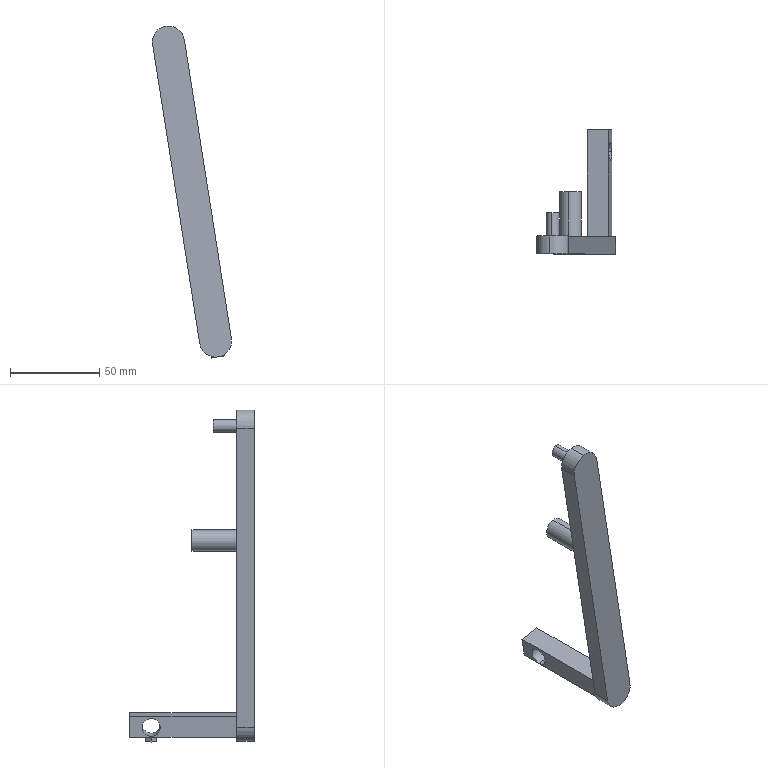Component | SolidWorks | Part2-1 | 1 solid | 27 faces | box 44.44 x 70 x 186.41 mm | volume 44277 mm3 | plane 18 | cylinder 9 | commonest cylinder face diameters 18 x3 10.1 x2 12 x2 7.1 x2
build123d program:
from build123d import *

# Parameters (mm, degrees)
SKETCH1_2_R         = 6
BOSS_EXTRUDE1_DEPTH = 10
SKETCH2_R           = 3.55
BOSS_EXTRUDE2_DEPTH = 13
SKETCH3_R           = 6
BOSS_EXTRUDE3_DEPTH = 25
SKETCH5_R           = 6
BOSS_EXTRUDE5_DEPTH = 20
SKETCH6_W           = 12
SKETCH6_H           = 12
BOSS_EXTRUDE6_DEPTH = 60
BOSS_EXTRUDE7_DEPTH = 3
SKETCH1_R           = 5.05
CUT_EXTRUDE1_DEPTH  = 193.785


with BuildPart() as part:
    # Sketch1_2 → Boss-Extrude1 (new body)
    with BuildSketch(Plane(origin=(0, 0, 0), x_dir=(0, 0, -1), z_dir=(1, 0, 0))):
        with BuildLine():
            Line((0, 9), (170, 9))
            ThreePointArc((170, 9), (179, 0), (170, -9))
            Line((170, -9), (0, -9))
            ThreePointArc((0, -9), (-9, 0), (0, 9))
        make_face()
        with Locations((65, 0)):
            Circle(SKETCH1_2_R, mode=Mode.SUBTRACT)
    extrude(amount=BOSS_EXTRUDE1_DEPTH)

    # Sketch2 → Boss-Extrude2 (add)
    with BuildSketch(Plane(origin=(10, 0, 0), x_dir=(0, 0, -1), z_dir=(1, 0, 0))):
        with Locations(Location((0, 0, 0), (0, 0, 180))):
            Circle(SKETCH2_R)
    extrude(amount=BOSS_EXTRUDE2_DEPTH)



with BuildPart() as body_2:
    # Sketch3 → Boss-Extrude3 (new body)
    with BuildSketch(Plane(origin=(10, 0, 0), x_dir=(0, 0, -1), z_dir=(1, 0, 0))):
        with Locations((65, 0)):
            Circle(SKETCH3_R)
    extrude(amount=BOSS_EXTRUDE3_DEPTH)


with BuildPart() as part_1:
    add(part.part)

    add(body_2.part)  # Boss-Extrude5 merges body 2
    # Sketch5 → Boss-Extrude5 (add)
    with BuildSketch(Plane.ZY):
        with Locations(Location((-65, 0, 0), (0, 0, 180))):
            Circle(SKETCH5_R)
    extrude(amount=-BOSS_EXTRUDE5_DEPTH)

    # Sketch6 → Boss-Extrude6 (add)
    with BuildSketch(Plane(origin=(10, 0, 0), x_dir=(0, 0, -1), z_dir=(1, 0, 0))):
        with Locations((170, 0)):
            Rectangle(SKETCH6_W, SKETCH6_H)
    extrude(amount=BOSS_EXTRUDE6_DEPTH)

    # Sketch7 → Boss-Extrude7 (add)
    with BuildSketch(Plane(origin=(0, 0, -176), x_dir=(-1, 0, 0), z_dir=(0, 0, -1))):
        Polygon((-58, -3.779), (-54.728, -1.889), (-54.728, 1.889), (-58, 3.779), (-61.272, 1.889), (-61.272, -1.889), align=None)
    extrude(amount=BOSS_EXTRUDE7_DEPTH)

    # Sketch1 → Cut-Extrude1 (cut, through all)
    with BuildSketch(Plane.XZ.offset(6)):
        with Locations(Location((57.862, -170.453, 0), (0, 0, 270))):
            Circle(SKETCH1_R)
    extrude(amount=-CUT_EXTRUDE1_DEPTH, mode=Mode.SUBTRACT)


solid = part_1.part

# Placed as in the assembly
solid = solid.moved(Location((679.123, -42.052, -108.622), (0, -8.948, 90)))
STEP:
#1=COLOUR_RGB('',0.7922,0.8196,0.9333);
#2=FILL_AREA_STYLE_COLOUR('',#1);
#3=FILL_AREA_STYLE('',(#2));
#4=SURFACE_STYLE_FILL_AREA(#3);
#5=SURFACE_SIDE_STYLE('',(#4));
#6=SURFACE_STYLE_USAGE(.BOTH.,#5);
#7=PRESENTATION_STYLE_ASSIGNMENT((#6));
#8=CARTESIAN_POINT('',(27.517,0.6224,-10.746));
#9=VERTEX_POINT('',#8);
#10=CARTESIAN_POINT('',(27.578,0.6224,-11.139));
#11=VERTEX_POINT('',#10);
#12=CARTESIAN_POINT('',(27.548,0.6224,-10.942));
#13=DIRECTION('',(0.9878,-0.,0.1555));
#14=DIRECTION('',(0.1555,0.,-0.9878));
#15=AXIS2_PLACEMENT_3D('',#12,#13,#14);
#16=CIRCLE('',#15,0.1988);
#17=EDGE_CURVE('',#9,#11,#16,.T.);
#18=ORIENTED_EDGE('',*,*,#17,.F.);
#19=CARTESIAN_POINT('',(27.983,0.6224,-10.672));
#20=VERTEX_POINT('',#19);
#21=CARTESIAN_POINT('',(27.4,0.6224,-10.764));
#22=DIRECTION('',(0.9878,-0.,0.1555));
#23=VECTOR('',#22,39.37);
#24=LINE('',#21,#23);
#25=EDGE_CURVE('',#9,#20,#24,.T.);
#26=ORIENTED_EDGE('',*,*,#25,.T.);
#27=CARTESIAN_POINT('',(28.045,0.6224,-11.065));
#28=VERTEX_POINT('',#27);
#29=CARTESIAN_POINT('',(28.014,0.6224,-10.869));
#30=DIRECTION('',(0.9878,-0.,0.1555));
#31=DIRECTION('',(0.1555,0.,-0.9878));
#32=AXIS2_PLACEMENT_3D('',#29,#30,#31);
#33=CIRCLE('',#32,0.1988);
#34=EDGE_CURVE('',#20,#28,#33,.T.);
#35=ORIENTED_EDGE('',*,*,#34,.T.);
#36=CARTESIAN_POINT('',(27.462,0.6224,-11.157));
#37=DIRECTION('',(0.9878,-0.,0.1555));
#38=VECTOR('',#37,39.37);
#39=LINE('',#36,#38);
#40=EDGE_CURVE('',#11,#28,#39,.T.);
#41=ORIENTED_EDGE('',*,*,#40,.F.);
#42=EDGE_LOOP('',(#18,#26,#35,#41));
#43=FACE_OUTER_BOUND('',#42,.T.);
#44=CARTESIAN_POINT('',(27.431,0.6224,-10.961));
#45=DIRECTION('',(0.9878,-0.,0.1555));
#46=DIRECTION('',(0.1555,0.,-0.9878));
#47=AXIS2_PLACEMENT_3D('',#44,#45,#46);
#48=CYLINDRICAL_SURFACE('',#47,0.1988);
#49=ADVANCED_FACE('',(#43),#48,.F.);
#50=CARTESIAN_POINT('',(27.172,-0.2776,-7.038));
#51=VERTEX_POINT('',#50);
#52=CARTESIAN_POINT('',(27.098,-0.2776,-6.571));
#53=VERTEX_POINT('',#52);
#54=CARTESIAN_POINT('',(27.135,-0.2776,-6.804));
#55=DIRECTION('',(0.,1.,0.));
#56=DIRECTION('',(0.1555,0.,-0.9878));
#57=AXIS2_PLACEMENT_3D('',#54,#55,#56);
#58=CIRCLE('',#57,0.2362);
#59=EDGE_CURVE('',#51,#53,#58,.T.);
#60=ORIENTED_EDGE('',*,*,#59,.F.);
#61=CARTESIAN_POINT('',(27.172,-1.262,-7.038));
#62=VERTEX_POINT('',#61);
#63=CARTESIAN_POINT('',(27.172,-0.8682,-7.038));
#64=DIRECTION('',(-0.,-1.,-0.));
#65=VECTOR('',#64,39.37);
#66=LINE('',#63,#65);
#67=EDGE_CURVE('',#51,#62,#66,.T.);
#68=ORIENTED_EDGE('',*,*,#67,.T.);
#69=CARTESIAN_POINT('',(27.098,-1.262,-6.571));
#70=VERTEX_POINT('',#69);
#71=CARTESIAN_POINT('',(27.135,-1.262,-6.804));
#72=DIRECTION('',(0.,1.,0.));
#73=DIRECTION('',(0.1555,0.,-0.9878));
#74=AXIS2_PLACEMENT_3D('',#71,#72,#73);
#75=CIRCLE('',#74,0.2362);
#76=EDGE_CURVE('',#62,#70,#75,.T.);
#77=ORIENTED_EDGE('',*,*,#76,.T.);
#78=CARTESIAN_POINT('',(27.098,-0.8682,-6.571));
#79=DIRECTION('',(-0.,-1.,-0.));
#80=VECTOR('',#79,39.37);
#81=LINE('',#78,#80);
#82=EDGE_CURVE('',#53,#70,#81,.T.);
#83=ORIENTED_EDGE('',*,*,#82,.F.);
#84=EDGE_LOOP('',(#60,#68,#77,#83));
#85=FACE_OUTER_BOUND('',#84,.T.);
#86=CARTESIAN_POINT('',(27.135,-0.8682,-6.804));
#87=DIRECTION('',(-0.,-1.,-0.));
#88=DIRECTION('',(-0.1555,0.,0.9878));
#89=AXIS2_PLACEMENT_3D('',#86,#87,#88);
#90=CYLINDRICAL_SURFACE('',#89,0.2362);
#91=ADVANCED_FACE('',(#85),#90,.T.);
#92=CARTESIAN_POINT('',(26.759,-0.7501,-4.415));
#93=VERTEX_POINT('',#92);
#94=CARTESIAN_POINT('',(26.715,-0.7501,-4.138));
#95=VERTEX_POINT('',#94);
#96=CARTESIAN_POINT('',(26.737,-0.7501,-4.276));
#97=DIRECTION('',(0.,1.,0.));
#98=DIRECTION('',(0.1555,0.,-0.9878));
#99=AXIS2_PLACEMENT_3D('',#96,#97,#98);
#100=CIRCLE('',#99,0.1398);
#101=EDGE_CURVE('',#93,#95,#100,.T.);
#102=ORIENTED_EDGE('',*,*,#101,.F.);
#103=CARTESIAN_POINT('',(26.759,-1.262,-4.415));
#104=VERTEX_POINT('',#103);
#105=CARTESIAN_POINT('',(26.759,-0.7501,-4.415));
#106=DIRECTION('',(-0.,-1.,-0.));
#107=VECTOR('',#106,39.37);
#108=LINE('',#105,#107);
#109=EDGE_CURVE('',#93,#104,#108,.T.);
#110=ORIENTED_EDGE('',*,*,#109,.T.);
#111=CARTESIAN_POINT('',(26.715,-1.262,-4.138));
#112=VERTEX_POINT('',#111);
#113=CARTESIAN_POINT('',(26.737,-1.262,-4.276));
#114=DIRECTION('',(0.,1.,0.));
#115=DIRECTION('',(0.1555,0.,-0.9878));
#116=AXIS2_PLACEMENT_3D('',#113,#114,#115);
#117=CIRCLE('',#116,0.1398);
#118=EDGE_CURVE('',#104,#112,#117,.T.);
#119=ORIENTED_EDGE('',*,*,#118,.T.);
#120=CARTESIAN_POINT('',(26.715,-0.7501,-4.138));
#121=DIRECTION('',(-0.,-1.,-0.));
#122=VECTOR('',#121,39.37);
#123=LINE('',#120,#122);
#124=EDGE_CURVE('',#95,#112,#123,.T.);
#125=ORIENTED_EDGE('',*,*,#124,.F.);
#126=EDGE_LOOP('',(#102,#110,#119,#125));
#127=FACE_OUTER_BOUND('',#126,.T.);
#128=CARTESIAN_POINT('',(26.737,-0.7501,-4.276));
#129=DIRECTION('',(-0.,-1.,-0.));
#130=DIRECTION('',(-0.1555,0.,0.9878));
#131=AXIS2_PLACEMENT_3D('',#128,#129,#130);
#132=CYLINDRICAL_SURFACE('',#131,0.1398);
#133=ADVANCED_FACE('',(#127),#132,.T.);
#134=CARTESIAN_POINT('',(26.682,-1.262,-3.926));
#135=VERTEX_POINT('',#134);
#136=CARTESIAN_POINT('',(27.087,-1.262,-4.221));
#137=VERTEX_POINT('',#136);
#138=CARTESIAN_POINT('',(26.737,-1.262,-4.276));
#139=DIRECTION('',(0.,1.,0.));
#140=DIRECTION('',(0.1555,0.,-0.9878));
#141=AXIS2_PLACEMENT_3D('',#138,#139,#140);
#142=CIRCLE('',#141,0.3543);
#143=EDGE_CURVE('',#135,#137,#142,.T.);
#144=ORIENTED_EDGE('',*,*,#143,.F.);
#145=CARTESIAN_POINT('',(26.682,-1.656,-3.926));
#146=VERTEX_POINT('',#145);
#147=CARTESIAN_POINT('',(26.682,-1.262,-3.926));
#148=DIRECTION('',(-0.,-1.,-0.));
#149=VECTOR('',#148,39.37);
#150=LINE('',#147,#149);
#151=EDGE_CURVE('',#135,#146,#150,.T.);
#152=ORIENTED_EDGE('',*,*,#151,.T.);
#153=CARTESIAN_POINT('',(27.087,-1.656,-4.221));
#154=VERTEX_POINT('',#153);
#155=CARTESIAN_POINT('',(26.737,-1.656,-4.276));
#156=DIRECTION('',(0.,1.,0.));
#157=DIRECTION('',(0.1555,0.,-0.9878));
#158=AXIS2_PLACEMENT_3D('',#155,#156,#157);
#159=CIRCLE('',#158,0.3543);
#160=EDGE_CURVE('',#146,#154,#159,.T.);
#161=ORIENTED_EDGE('',*,*,#160,.T.);
#162=CARTESIAN_POINT('',(27.087,-1.262,-4.221));
#163=DIRECTION('',(-0.,-1.,-0.));
#164=VECTOR('',#163,39.37);
#165=LINE('',#162,#164);
#166=EDGE_CURVE('',#137,#154,#165,.T.);
#167=ORIENTED_EDGE('',*,*,#166,.F.);
#168=EDGE_LOOP('',(#144,#152,#161,#167));
#169=FACE_OUTER_BOUND('',#168,.T.);
#170=CARTESIAN_POINT('',(26.737,-1.262,-4.276));
#171=DIRECTION('',(-0.,-1.,-0.));
#172=DIRECTION('',(-0.1555,0.,0.9878));
#173=AXIS2_PLACEMENT_3D('',#170,#171,#172);
#174=CYLINDRICAL_SURFACE('',#173,0.3543);
#175=ADVANCED_FACE('',(#169),#174,.T.);
#176=CARTESIAN_POINT('',(28.048,-1.262,-11.085));
#177=VERTEX_POINT('',#176);
#178=CARTESIAN_POINT('',(27.581,-1.262,-11.158));
#179=VERTEX_POINT('',#178);
#180=CARTESIAN_POINT('',(27.581,-1.262,-11.158));
#181=DIRECTION('',(-0.9878,0.,-0.1555));
#182=VECTOR('',#181,39.37);
#183=LINE('',#180,#182);
#184=EDGE_CURVE('',#177,#179,#183,.T.);
#185=ORIENTED_EDGE('',*,*,#184,.T.);
#186=CARTESIAN_POINT('',(27.581,1.1,-11.158));
#187=VERTEX_POINT('',#186);
#188=CARTESIAN_POINT('',(27.581,1.1,-11.158));
#189=DIRECTION('',(-0.,-1.,-0.));
#190=VECTOR('',#189,39.37);
#191=LINE('',#188,#190);
#192=EDGE_CURVE('',#187,#179,#191,.T.);
#193=ORIENTED_EDGE('',*,*,#192,.F.);
#194=CARTESIAN_POINT('',(28.048,1.1,-11.085));
#195=VERTEX_POINT('',#194);
#196=CARTESIAN_POINT('',(27.581,1.1,-11.158));
#197=DIRECTION('',(-0.9878,0.,-0.1555));
#198=VECTOR('',#197,39.37);
#199=LINE('',#196,#198);
#200=EDGE_CURVE('',#195,#187,#199,.T.);
#201=ORIENTED_EDGE('',*,*,#200,.F.);
#202=CARTESIAN_POINT('',(28.048,1.1,-11.085));
#203=DIRECTION('',(-0.,-1.,-0.));
#204=VECTOR('',#203,39.37);
#205=LINE('',#202,#204);
#206=EDGE_CURVE('',#195,#177,#205,.T.);
#207=ORIENTED_EDGE('',*,*,#206,.T.);
#208=EDGE_LOOP('',(#185,#193,#201,#207));
#209=FACE_OUTER_BOUND('',#208,.T.);
#210=CARTESIAN_POINT('',(27.888,0.7567,-11.11));
#211=VERTEX_POINT('',#210);
#212=CARTESIAN_POINT('',(27.962,0.6279,-11.098));
#213=VERTEX_POINT('',#212);
#214=CARTESIAN_POINT('',(27.888,0.7567,-11.11));
#215=DIRECTION('',(0.4939,-0.866,0.07776));
#216=VECTOR('',#215,39.37);
#217=LINE('',#214,#216);
#218=EDGE_CURVE('',#211,#213,#217,.T.);
#219=ORIENTED_EDGE('',*,*,#218,.F.);
#220=CARTESIAN_POINT('',(27.741,0.7567,-11.133));
#221=VERTEX_POINT('',#220);
#222=CARTESIAN_POINT('',(27.741,0.7567,-11.133));
#223=DIRECTION('',(0.9878,-0.,0.1555));
#224=VECTOR('',#223,39.37);
#225=LINE('',#222,#224);
#226=EDGE_CURVE('',#221,#211,#225,.T.);
#227=ORIENTED_EDGE('',*,*,#226,.F.);
#228=CARTESIAN_POINT('',(27.668,0.6279,-11.144));
#229=VERTEX_POINT('',#228);
#230=CARTESIAN_POINT('',(27.668,0.6279,-11.144));
#231=DIRECTION('',(0.4939,0.866,0.07776));
#232=VECTOR('',#231,39.37);
#233=LINE('',#230,#232);
#234=EDGE_CURVE('',#229,#221,#233,.T.);
#235=ORIENTED_EDGE('',*,*,#234,.F.);
#236=CARTESIAN_POINT('',(27.741,0.499,-11.133));
#237=VERTEX_POINT('',#236);
#238=CARTESIAN_POINT('',(27.741,0.499,-11.133));
#239=DIRECTION('',(-0.4939,0.866,-0.07776));
#240=VECTOR('',#239,39.37);
#241=LINE('',#238,#240);
#242=EDGE_CURVE('',#237,#229,#241,.T.);
#243=ORIENTED_EDGE('',*,*,#242,.F.);
#244=CARTESIAN_POINT('',(27.888,0.499,-11.11));
#245=VERTEX_POINT('',#244);
#246=CARTESIAN_POINT('',(27.888,0.499,-11.11));
#247=DIRECTION('',(-0.9878,0.,-0.1555));
#248=VECTOR('',#247,39.37);
#249=LINE('',#246,#248);
#250=EDGE_CURVE('',#245,#237,#249,.T.);
#251=ORIENTED_EDGE('',*,*,#250,.F.);
#252=CARTESIAN_POINT('',(27.962,0.6279,-11.098));
#253=DIRECTION('',(-0.4939,-0.866,-0.07776));
#254=VECTOR('',#253,39.37);
#255=LINE('',#252,#254);
#256=EDGE_CURVE('',#213,#245,#255,.T.);
#257=ORIENTED_EDGE('',*,*,#256,.F.);
#258=EDGE_LOOP('',(#219,#227,#235,#243,#251,#257));
#259=FACE_BOUND('',#258,.T.);
#260=CARTESIAN_POINT('',(27.581,1.1,-11.158));
#261=DIRECTION('',(-0.1555,0.,0.9878));
#262=DIRECTION('',(0.,1.,0.));
#263=AXIS2_PLACEMENT_3D('',#260,#261,#262);
#264=PLANE('',#263);
#265=ADVANCED_FACE('',(#209,#259),#264,.F.);
#266=CARTESIAN_POINT('',(27.135,-1.262,-6.804));
#267=DIRECTION('',(0.,1.,0.));
#268=DIRECTION('',(0.1555,0.,-0.9878));
#269=AXIS2_PLACEMENT_3D('',#266,#267,#268);
#270=CIRCLE('',#269,0.2362);
#271=EDGE_CURVE('',#70,#62,#270,.T.);
#272=ORIENTED_EDGE('',*,*,#271,.F.);
#273=ORIENTED_EDGE('',*,*,#76,.F.);
#274=EDGE_LOOP('',(#272,#273));
#275=FACE_BOUND('',#274,.T.);
#276=CARTESIAN_POINT('',(26.387,-1.262,-4.332));
#277=VERTEX_POINT('',#276);
#278=CARTESIAN_POINT('',(26.737,-1.262,-4.276));
#279=DIRECTION('',(0.,1.,0.));
#280=DIRECTION('',(0.1555,0.,-0.9878));
#281=AXIS2_PLACEMENT_3D('',#278,#279,#280);
#282=CIRCLE('',#281,0.3543);
#283=EDGE_CURVE('',#277,#135,#282,.T.);
#284=ORIENTED_EDGE('',*,*,#283,.T.);
#285=ORIENTED_EDGE('',*,*,#143,.T.);
#286=CARTESIAN_POINT('',(28.128,-1.262,-10.833));
#287=VERTEX_POINT('',#286);
#288=CARTESIAN_POINT('',(27.087,-1.262,-4.221));
#289=DIRECTION('',(0.1555,-0.,-0.9878));
#290=VECTOR('',#289,39.37);
#291=LINE('',#288,#290);
#292=EDGE_CURVE('',#137,#287,#291,.T.);
#293=ORIENTED_EDGE('',*,*,#292,.T.);
#294=CARTESIAN_POINT('',(27.428,-1.262,-10.943));
#295=VERTEX_POINT('',#294);
#296=CARTESIAN_POINT('',(27.778,-1.262,-10.888));
#297=DIRECTION('',(0.,1.,0.));
#298=DIRECTION('',(0.1555,0.,-0.9878));
#299=AXIS2_PLACEMENT_3D('',#296,#297,#298);
#300=CIRCLE('',#299,0.3543);
#301=EDGE_CURVE('',#287,#295,#300,.T.);
#302=ORIENTED_EDGE('',*,*,#301,.T.);
#303=CARTESIAN_POINT('',(26.387,-1.262,-4.332));
#304=DIRECTION('',(-0.1555,0.,0.9878));
#305=VECTOR('',#304,39.37);
#306=LINE('',#303,#305);
#307=EDGE_CURVE('',#295,#277,#306,.T.);
#308=ORIENTED_EDGE('',*,*,#307,.T.);
#309=EDGE_LOOP('',(#284,#285,#293,#302,#308));
#310=FACE_OUTER_BOUND('',#309,.T.);
#311=CARTESIAN_POINT('',(26.737,-1.262,-4.276));
#312=DIRECTION('',(0.,1.,0.));
#313=DIRECTION('',(0.1555,0.,-0.9878));
#314=AXIS2_PLACEMENT_3D('',#311,#312,#313);
#315=CIRCLE('',#314,0.1398);
#316=EDGE_CURVE('',#112,#104,#315,.T.);
#317=ORIENTED_EDGE('',*,*,#316,.F.);
#318=ORIENTED_EDGE('',*,*,#118,.F.);
#319=EDGE_LOOP('',(#317,#318));
#320=FACE_BOUND('',#319,.T.);
#321=CARTESIAN_POINT('',(27.975,-1.262,-10.618));
#322=VERTEX_POINT('',#321);
#323=CARTESIAN_POINT('',(28.048,-1.262,-11.085));
#324=DIRECTION('',(0.1555,-0.,-0.9878));
#325=VECTOR('',#324,39.37);
#326=LINE('',#323,#325);
#327=EDGE_CURVE('',#322,#177,#326,.T.);
#328=ORIENTED_EDGE('',*,*,#327,.F.);
#329=CARTESIAN_POINT('',(27.508,-1.262,-10.691));
#330=VERTEX_POINT('',#329);
#331=CARTESIAN_POINT('',(27.508,-1.262,-10.691));
#332=DIRECTION('',(0.9878,-0.,0.1555));
#333=VECTOR('',#332,39.37);
#334=LINE('',#331,#333);
#335=EDGE_CURVE('',#330,#322,#334,.T.);
#336=ORIENTED_EDGE('',*,*,#335,.F.);
#337=CARTESIAN_POINT('',(27.581,-1.262,-11.158));
#338=DIRECTION('',(-0.1555,0.,0.9878));
#339=VECTOR('',#338,39.37);
#340=LINE('',#337,#339);
#341=EDGE_CURVE('',#179,#330,#340,.T.);
#342=ORIENTED_EDGE('',*,*,#341,.F.);
#343=ORIENTED_EDGE('',*,*,#184,.F.);
#344=EDGE_LOOP('',(#328,#336,#342,#343));
#345=FACE_BOUND('',#344,.T.);
#346=CARTESIAN_POINT('',(26.737,-1.262,-4.276));
#347=DIRECTION('',(0.,1.,0.));
#348=DIRECTION('',(0.1555,-0.,-0.9878));
#349=AXIS2_PLACEMENT_3D('',#346,#347,#348);
#350=PLANE('',#349);
#351=ADVANCED_FACE('',(#275,#310,#320,#345),#350,.T.);
#352=CARTESIAN_POINT('',(26.387,-1.656,-4.332));
#353=VERTEX_POINT('',#352);
#354=CARTESIAN_POINT('',(26.737,-1.656,-4.276));
#355=DIRECTION('',(0.,1.,0.));
#356=DIRECTION('',(0.1555,0.,-0.9878));
#357=AXIS2_PLACEMENT_3D('',#354,#355,#356);
#358=CIRCLE('',#357,0.3543);
#359=EDGE_CURVE('',#353,#146,#358,.T.);
#360=ORIENTED_EDGE('',*,*,#359,.F.);
#361=CARTESIAN_POINT('',(27.428,-1.656,-10.943));
#362=VERTEX_POINT('',#361);
#363=CARTESIAN_POINT('',(26.387,-1.656,-4.332));
#364=DIRECTION('',(-0.1555,0.,0.9878));
#365=VECTOR('',#364,39.37);
#366=LINE('',#363,#365);
#367=EDGE_CURVE('',#362,#353,#366,.T.);
#368=ORIENTED_EDGE('',*,*,#367,.F.);
#369=CARTESIAN_POINT('',(28.128,-1.656,-10.833));
#370=VERTEX_POINT('',#369);
#371=CARTESIAN_POINT('',(27.778,-1.656,-10.888));
#372=DIRECTION('',(0.,1.,0.));
#373=DIRECTION('',(0.1555,0.,-0.9878));
#374=AXIS2_PLACEMENT_3D('',#371,#372,#373);
#375=CIRCLE('',#374,0.3543);
#376=EDGE_CURVE('',#370,#362,#375,.T.);
#377=ORIENTED_EDGE('',*,*,#376,.F.);
#378=CARTESIAN_POINT('',(27.087,-1.656,-4.221));
#379=DIRECTION('',(0.1555,-0.,-0.9878));
#380=VECTOR('',#379,39.37);
#381=LINE('',#378,#380);
#382=EDGE_CURVE('',#154,#370,#381,.T.);
#383=ORIENTED_EDGE('',*,*,#382,.F.);
#384=ORIENTED_EDGE('',*,*,#160,.F.);
#385=EDGE_LOOP('',(#360,#368,#377,#383,#384));
#386=FACE_OUTER_BOUND('',#385,.T.);
#387=CARTESIAN_POINT('',(26.737,-1.656,-4.276));
#388=DIRECTION('',(0.,1.,0.));
#389=DIRECTION('',(0.1555,-0.,-0.9878));
#390=AXIS2_PLACEMENT_3D('',#387,#388,#389);
#391=PLANE('',#390);
#392=ADVANCED_FACE('',(#386),#391,.F.);
#393=ORIENTED_EDGE('',*,*,#151,.F.);
#394=ORIENTED_EDGE('',*,*,#283,.F.);
#395=CARTESIAN_POINT('',(26.387,-1.262,-4.332));
#396=DIRECTION('',(-0.,-1.,-0.));
#397=VECTOR('',#396,39.37);
#398=LINE('',#395,#397);
#399=EDGE_CURVE('',#277,#353,#398,.T.);
#400=ORIENTED_EDGE('',*,*,#399,.T.);
#401=ORIENTED_EDGE('',*,*,#359,.T.);
#402=EDGE_LOOP('',(#393,#394,#400,#401));
#403=FACE_OUTER_BOUND('',#402,.T.);
#404=CARTESIAN_POINT('',(26.737,-1.262,-4.276));
#405=DIRECTION('',(-0.,-1.,-0.));
#406=DIRECTION('',(-0.1555,0.,0.9878));
#407=AXIS2_PLACEMENT_3D('',#404,#405,#406);
#408=CYLINDRICAL_SURFACE('',#407,0.3543);
#409=ADVANCED_FACE('',(#403),#408,.T.);
#410=ORIENTED_EDGE('',*,*,#382,.T.);
#411=CARTESIAN_POINT('',(28.128,-1.262,-10.833));
#412=DIRECTION('',(-0.,-1.,-0.));
#413=VECTOR('',#412,39.37);
#414=LINE('',#411,#413);
#415=EDGE_CURVE('',#287,#370,#414,.T.);
#416=ORIENTED_EDGE('',*,*,#415,.F.);
#417=ORIENTED_EDGE('',*,*,#292,.F.);
#418=ORIENTED_EDGE('',*,*,#166,.T.);
#419=EDGE_LOOP('',(#410,#416,#417,#418));
#420=FACE_OUTER_BOUND('',#419,.T.);
#421=CARTESIAN_POINT('',(27.087,-1.262,-4.221));
#422=DIRECTION('',(-0.9878,0.,-0.1555));
#423=DIRECTION('',(-0.1555,0.,0.9878));
#424=AXIS2_PLACEMENT_3D('',#421,#422,#423);
#425=PLANE('',#424);
#426=ADVANCED_FACE('',(#420),#425,.F.);
#427=ORIENTED_EDGE('',*,*,#376,.T.);
#428=CARTESIAN_POINT('',(27.428,-1.262,-10.943));
#429=DIRECTION('',(-0.,-1.,-0.));
#430=VECTOR('',#429,39.37);
#431=LINE('',#428,#430);
#432=EDGE_CURVE('',#295,#362,#431,.T.);
#433=ORIENTED_EDGE('',*,*,#432,.F.);
#434=ORIENTED_EDGE('',*,*,#301,.F.);
#435=ORIENTED_EDGE('',*,*,#415,.T.);
#436=EDGE_LOOP('',(#427,#433,#434,#435));
#437=FACE_OUTER_BOUND('',#436,.T.);
#438=CARTESIAN_POINT('',(27.778,-1.262,-10.888));
#439=DIRECTION('',(-0.,-1.,-0.));
#440=DIRECTION('',(-0.1555,0.,0.9878));
#441=AXIS2_PLACEMENT_3D('',#438,#439,#440);
#442=CYLINDRICAL_SURFACE('',#441,0.3543);
#443=ADVANCED_FACE('',(#437),#442,.T.);
#444=ORIENTED_EDGE('',*,*,#367,.T.);
#445=ORIENTED_EDGE('',*,*,#399,.F.);
#446=ORIENTED_EDGE('',*,*,#307,.F.);
#447=ORIENTED_EDGE('',*,*,#432,.T.);
#448=EDGE_LOOP('',(#444,#445,#446,#447));
#449=FACE_OUTER_BOUND('',#448,.T.);
#450=CARTESIAN_POINT('',(26.387,-1.262,-4.332));
#451=DIRECTION('',(0.9878,-0.,0.1555));
#452=DIRECTION('',(0.1555,-0.,-0.9878));
#453=AXIS2_PLACEMENT_3D('',#450,#451,#452);
#454=PLANE('',#453);
#455=ADVANCED_FACE('',(#449),#454,.F.);
#456=ORIENTED_EDGE('',*,*,#109,.F.);
#457=CARTESIAN_POINT('',(26.737,-0.7501,-4.276));
#458=DIRECTION('',(0.,1.,0.));
#459=DIRECTION('',(0.1555,0.,-0.9878));
#460=AXIS2_PLACEMENT_3D('',#457,#458,#459);
#461=CIRCLE('',#460,0.1398);
#462=EDGE_CURVE('',#95,#93,#461,.T.);
#463=ORIENTED_EDGE('',*,*,#462,.F.);
#464=ORIENTED_EDGE('',*,*,#124,.T.);
#465=ORIENTED_EDGE('',*,*,#316,.T.);
#466=EDGE_LOOP('',(#456,#463,#464,#465));
#467=FACE_OUTER_BOUND('',#466,.T.);
#468=CARTESIAN_POINT('',(26.737,-0.7501,-4.276));
#469=DIRECTION('',(-0.,-1.,-0.));
#470=DIRECTION('',(-0.1555,0.,0.9878));
#471=AXIS2_PLACEMENT_3D('',#468,#469,#470);
#472=CYLINDRICAL_SURFACE('',#471,0.1398);
#473=ADVANCED_FACE('',(#467),#472,.T.);
#474=ORIENTED_EDGE('',*,*,#462,.T.);
#475=ORIENTED_EDGE('',*,*,#101,.T.);
#476=EDGE_LOOP('',(#474,#475));
#477=FACE_OUTER_BOUND('',#476,.T.);
#478=CARTESIAN_POINT('',(26.737,-0.7501,-4.276));
#479=DIRECTION('',(0.,1.,0.));
#480=DIRECTION('',(0.1555,-0.,-0.9878));
#481=AXIS2_PLACEMENT_3D('',#478,#479,#480);
#482=PLANE('',#481);
#483=ADVANCED_FACE('',(#477),#482,.T.);
#484=ORIENTED_EDGE('',*,*,#67,.F.);
#485=CARTESIAN_POINT('',(27.135,-0.2776,-6.804));
#486=DIRECTION('',(0.,1.,0.));
#487=DIRECTION('',(0.1555,0.,-0.9878));
#488=AXIS2_PLACEMENT_3D('',#485,#486,#487);
#489=CIRCLE('',#488,0.2362);
#490=EDGE_CURVE('',#53,#51,#489,.T.);
#491=ORIENTED_EDGE('',*,*,#490,.F.);
#492=ORIENTED_EDGE('',*,*,#82,.T.);
#493=ORIENTED_EDGE('',*,*,#271,.T.);
#494=EDGE_LOOP('',(#484,#491,#492,#493));
#495=FACE_OUTER_BOUND('',#494,.T.);
#496=CARTESIAN_POINT('',(27.135,-0.8682,-6.804));
#497=DIRECTION('',(-0.,-1.,-0.));
#498=DIRECTION('',(-0.1555,0.,0.9878));
#499=AXIS2_PLACEMENT_3D('',#496,#497,#498);
#500=CYLINDRICAL_SURFACE('',#499,0.2362);
#501=ADVANCED_FACE('',(#495),#500,.T.);
#502=ORIENTED_EDGE('',*,*,#490,.T.);
#503=ORIENTED_EDGE('',*,*,#59,.T.);
#504=EDGE_LOOP('',(#502,#503));
#505=FACE_OUTER_BOUND('',#504,.T.);
#506=CARTESIAN_POINT('',(27.135,-0.2776,-6.804));
#507=DIRECTION('',(0.,1.,0.));
#508=DIRECTION('',(0.1555,-0.,-0.9878));
#509=AXIS2_PLACEMENT_3D('',#506,#507,#508);
#510=PLANE('',#509);
#511=ADVANCED_FACE('',(#505),#510,.T.);
#512=ORIENTED_EDGE('',*,*,#335,.T.);
#513=CARTESIAN_POINT('',(27.975,1.1,-10.618));
#514=VERTEX_POINT('',#513);
#515=CARTESIAN_POINT('',(27.975,1.1,-10.618));
#516=DIRECTION('',(-0.,-1.,-0.));
#517=VECTOR('',#516,39.37);
#518=LINE('',#515,#517);
#519=EDGE_CURVE('',#514,#322,#518,.T.);
#520=ORIENTED_EDGE('',*,*,#519,.F.);
#521=CARTESIAN_POINT('',(27.508,1.1,-10.691));
#522=VERTEX_POINT('',#521);
#523=CARTESIAN_POINT('',(27.508,1.1,-10.691));
#524=DIRECTION('',(0.9878,-0.,0.1555));
#525=VECTOR('',#524,39.37);
#526=LINE('',#523,#525);
#527=EDGE_CURVE('',#522,#514,#526,.T.);
#528=ORIENTED_EDGE('',*,*,#527,.F.);
#529=CARTESIAN_POINT('',(27.508,1.1,-10.691));
#530=DIRECTION('',(-0.,-1.,-0.));
#531=VECTOR('',#530,39.37);
#532=LINE('',#529,#531);
#533=EDGE_CURVE('',#522,#330,#532,.T.);
#534=ORIENTED_EDGE('',*,*,#533,.T.);
#535=EDGE_LOOP('',(#512,#520,#528,#534));
#536=FACE_OUTER_BOUND('',#535,.T.);
#537=CARTESIAN_POINT('',(27.508,1.1,-10.691));
#538=DIRECTION('',(0.1555,-0.,-0.9878));
#539=DIRECTION('',(-0.,-1.,-0.));
#540=AXIS2_PLACEMENT_3D('',#537,#538,#539);
#541=PLANE('',#540);
#542=ADVANCED_FACE('',(#536),#541,.F.);
#543=CARTESIAN_POINT('',(28.014,0.6224,-10.869));
#544=DIRECTION('',(0.9878,-0.,0.1555));
#545=DIRECTION('',(0.1555,0.,-0.9878));
#546=AXIS2_PLACEMENT_3D('',#543,#544,#545);
#547=CIRCLE('',#546,0.1988);
#548=EDGE_CURVE('',#28,#20,#547,.T.);
#549=ORIENTED_EDGE('',*,*,#548,.F.);
#550=ORIENTED_EDGE('',*,*,#34,.F.);
#551=EDGE_LOOP('',(#549,#550));
#552=FACE_BOUND('',#551,.T.);
#553=ORIENTED_EDGE('',*,*,#327,.T.);
#554=ORIENTED_EDGE('',*,*,#206,.F.);
#555=CARTESIAN_POINT('',(28.048,1.1,-11.085));
#556=DIRECTION('',(0.1555,-0.,-0.9878));
#557=VECTOR('',#556,39.37);
#558=LINE('',#555,#557);
#559=EDGE_CURVE('',#514,#195,#558,.T.);
#560=ORIENTED_EDGE('',*,*,#559,.F.);
#561=ORIENTED_EDGE('',*,*,#519,.T.);
#562=EDGE_LOOP('',(#553,#554,#560,#561));
#563=FACE_OUTER_BOUND('',#562,.T.);
#564=CARTESIAN_POINT('',(28.048,1.1,-11.085));
#565=DIRECTION('',(-0.9878,0.,-0.1555));
#566=DIRECTION('',(-0.1555,0.,0.9878));
#567=AXIS2_PLACEMENT_3D('',#564,#565,#566);
#568=PLANE('',#567);
#569=ADVANCED_FACE('',(#552,#563),#568,.F.);
#570=CARTESIAN_POINT('',(27.548,0.6224,-10.942));
#571=DIRECTION('',(0.9878,-0.,0.1555));
#572=DIRECTION('',(0.1555,0.,-0.9878));
#573=AXIS2_PLACEMENT_3D('',#570,#571,#572);
#574=CIRCLE('',#573,0.1988);
#575=EDGE_CURVE('',#11,#9,#574,.T.);
#576=ORIENTED_EDGE('',*,*,#575,.T.);
#577=ORIENTED_EDGE('',*,*,#17,.T.);
#578=EDGE_LOOP('',(#576,#577));
#579=FACE_BOUND('',#578,.T.);
#580=ORIENTED_EDGE('',*,*,#341,.T.);
#581=ORIENTED_EDGE('',*,*,#533,.F.);
#582=CARTESIAN_POINT('',(27.581,1.1,-11.158));
#583=DIRECTION('',(-0.1555,0.,0.9878));
#584=VECTOR('',#583,39.37);
#585=LINE('',#582,#584);
#586=EDGE_CURVE('',#187,#522,#585,.T.);
#587=ORIENTED_EDGE('',*,*,#586,.F.);
#588=ORIENTED_EDGE('',*,*,#192,.T.);
#589=EDGE_LOOP('',(#580,#581,#587,#588));
#590=FACE_OUTER_BOUND('',#589,.T.);
#591=CARTESIAN_POINT('',(27.581,1.1,-11.158));
#592=DIRECTION('',(0.9878,-0.,0.1555));
#593=DIRECTION('',(0.1555,-0.,-0.9878));
#594=AXIS2_PLACEMENT_3D('',#591,#592,#593);
#595=PLANE('',#594);
#596=ADVANCED_FACE('',(#579,#590),#595,.F.);
#597=ORIENTED_EDGE('',*,*,#527,.T.);
#598=ORIENTED_EDGE('',*,*,#559,.T.);
#599=ORIENTED_EDGE('',*,*,#200,.T.);
#600=ORIENTED_EDGE('',*,*,#586,.T.);
#601=EDGE_LOOP('',(#597,#598,#599,#600));
#602=FACE_OUTER_BOUND('',#601,.T.);
#603=CARTESIAN_POINT('',(26.737,1.1,-4.276));
#604=DIRECTION('',(-0.,-1.,-0.));
#605=DIRECTION('',(-0.1555,0.,0.9878));
#606=AXIS2_PLACEMENT_3D('',#603,#604,#605);
#607=PLANE('',#606);
#608=ADVANCED_FACE('',(#602),#607,.F.);
#609=ORIENTED_EDGE('',*,*,#218,.T.);
#610=CARTESIAN_POINT('',(27.98,0.6279,-11.215));
#611=VERTEX_POINT('',#610);
#612=CARTESIAN_POINT('',(27.98,0.6279,-11.215));
#613=DIRECTION('',(-0.1555,0.,0.9878));
#614=VECTOR('',#613,39.37);
#615=LINE('',#612,#614);
#616=EDGE_CURVE('',#611,#213,#615,.T.);
#617=ORIENTED_EDGE('',*,*,#616,.F.);
#618=CARTESIAN_POINT('',(27.907,0.7567,-11.226));
#619=VERTEX_POINT('',#618);
#620=CARTESIAN_POINT('',(27.907,0.7567,-11.226));
#621=DIRECTION('',(0.4939,-0.866,0.07776));
#622=VECTOR('',#621,39.37);
#623=LINE('',#620,#622);
#624=EDGE_CURVE('',#619,#611,#623,.T.);
#625=ORIENTED_EDGE('',*,*,#624,.F.);
#626=CARTESIAN_POINT('',(27.907,0.7567,-11.226));
#627=DIRECTION('',(-0.1555,0.,0.9878));
#628=VECTOR('',#627,39.37);
#629=LINE('',#626,#628);
#630=EDGE_CURVE('',#619,#211,#629,.T.);
#631=ORIENTED_EDGE('',*,*,#630,.T.);
#632=EDGE_LOOP('',(#609,#617,#625,#631));
#633=FACE_OUTER_BOUND('',#632,.T.);
#634=CARTESIAN_POINT('',(27.907,0.7567,-11.226));
#635=DIRECTION('',(-0.8555,-0.5,-0.1347));
#636=DIRECTION('',(0.4939,-0.866,0.07776));
#637=AXIS2_PLACEMENT_3D('',#634,#635,#636);
#638=PLANE('',#637);
#639=ADVANCED_FACE('',(#633),#638,.F.);
#640=ORIENTED_EDGE('',*,*,#256,.T.);
#641=CARTESIAN_POINT('',(27.907,0.499,-11.226));
#642=VERTEX_POINT('',#641);
#643=CARTESIAN_POINT('',(27.907,0.499,-11.226));
#644=DIRECTION('',(-0.1555,0.,0.9878));
#645=VECTOR('',#644,39.37);
#646=LINE('',#643,#645);
#647=EDGE_CURVE('',#642,#245,#646,.T.);
#648=ORIENTED_EDGE('',*,*,#647,.F.);
#649=CARTESIAN_POINT('',(27.98,0.6279,-11.215));
#650=DIRECTION('',(-0.4939,-0.866,-0.07776));
#651=VECTOR('',#650,39.37);
#652=LINE('',#649,#651);
#653=EDGE_CURVE('',#611,#642,#652,.T.);
#654=ORIENTED_EDGE('',*,*,#653,.F.);
#655=ORIENTED_EDGE('',*,*,#616,.T.);
#656=EDGE_LOOP('',(#640,#648,#654,#655));
#657=FACE_OUTER_BOUND('',#656,.T.);
#658=CARTESIAN_POINT('',(27.98,0.6279,-11.215));
#659=DIRECTION('',(-0.8555,0.5,-0.1347));
#660=DIRECTION('',(-0.4939,-0.866,-0.07776));
#661=AXIS2_PLACEMENT_3D('',#658,#659,#660);
#662=PLANE('',#661);
#663=ADVANCED_FACE('',(#657),#662,.F.);
#664=ORIENTED_EDGE('',*,*,#250,.T.);
#665=CARTESIAN_POINT('',(27.76,0.499,-11.25));
#666=VERTEX_POINT('',#665);
#667=CARTESIAN_POINT('',(27.76,0.499,-11.25));
#668=DIRECTION('',(-0.1555,0.,0.9878));
#669=VECTOR('',#668,39.37);
#670=LINE('',#667,#669);
#671=EDGE_CURVE('',#666,#237,#670,.T.);
#672=ORIENTED_EDGE('',*,*,#671,.F.);
#673=CARTESIAN_POINT('',(27.907,0.499,-11.226));
#674=DIRECTION('',(-0.9878,0.,-0.1555));
#675=VECTOR('',#674,39.37);
#676=LINE('',#673,#675);
#677=EDGE_CURVE('',#642,#666,#676,.T.);
#678=ORIENTED_EDGE('',*,*,#677,.F.);
#679=ORIENTED_EDGE('',*,*,#647,.T.);
#680=EDGE_LOOP('',(#664,#672,#678,#679));
#681=FACE_OUTER_BOUND('',#680,.T.);
#682=CARTESIAN_POINT('',(27.907,0.499,-11.226));
#683=DIRECTION('',(0.,1.,0.));
#684=DIRECTION('',(-0.9878,0.,-0.1555));
#685=AXIS2_PLACEMENT_3D('',#682,#683,#684);
#686=PLANE('',#685);
#687=ADVANCED_FACE('',(#681),#686,.F.);
#688=ORIENTED_EDGE('',*,*,#242,.T.);
#689=CARTESIAN_POINT('',(27.686,0.6279,-11.261));
#690=VERTEX_POINT('',#689);
#691=CARTESIAN_POINT('',(27.686,0.6279,-11.261));
#692=DIRECTION('',(-0.1555,0.,0.9878));
#693=VECTOR('',#692,39.37);
#694=LINE('',#691,#693);
#695=EDGE_CURVE('',#690,#229,#694,.T.);
#696=ORIENTED_EDGE('',*,*,#695,.F.);
#697=CARTESIAN_POINT('',(27.76,0.499,-11.25));
#698=DIRECTION('',(-0.4939,0.866,-0.07776));
#699=VECTOR('',#698,39.37);
#700=LINE('',#697,#699);
#701=EDGE_CURVE('',#666,#690,#700,.T.);
#702=ORIENTED_EDGE('',*,*,#701,.F.);
#703=ORIENTED_EDGE('',*,*,#671,.T.);
#704=EDGE_LOOP('',(#688,#696,#702,#703));
#705=FACE_OUTER_BOUND('',#704,.T.);
#706=CARTESIAN_POINT('',(27.76,0.499,-11.25));
#707=DIRECTION('',(0.8555,0.5,0.1347));
#708=DIRECTION('',(-0.4939,0.866,-0.07776));
#709=AXIS2_PLACEMENT_3D('',#706,#707,#708);
#710=PLANE('',#709);
#711=ADVANCED_FACE('',(#705),#710,.F.);
#712=ORIENTED_EDGE('',*,*,#234,.T.);
#713=CARTESIAN_POINT('',(27.76,0.7567,-11.25));
#714=VERTEX_POINT('',#713);
#715=CARTESIAN_POINT('',(27.76,0.7567,-11.25));
#716=DIRECTION('',(-0.1555,0.,0.9878));
#717=VECTOR('',#716,39.37);
#718=LINE('',#715,#717);
#719=EDGE_CURVE('',#714,#221,#718,.T.);
#720=ORIENTED_EDGE('',*,*,#719,.F.);
#721=CARTESIAN_POINT('',(27.686,0.6279,-11.261));
#722=DIRECTION('',(0.4939,0.866,0.07776));
#723=VECTOR('',#722,39.37);
#724=LINE('',#721,#723);
#725=EDGE_CURVE('',#690,#714,#724,.T.);
#726=ORIENTED_EDGE('',*,*,#725,.F.);
#727=ORIENTED_EDGE('',*,*,#695,.T.);
#728=EDGE_LOOP('',(#712,#720,#726,#727));
#729=FACE_OUTER_BOUND('',#728,.T.);
#730=CARTESIAN_POINT('',(27.686,0.6279,-11.261));
#731=DIRECTION('',(0.8555,-0.5,0.1347));
#732=DIRECTION('',(0.4939,0.866,0.07776));
#733=AXIS2_PLACEMENT_3D('',#730,#731,#732);
#734=PLANE('',#733);
#735=ADVANCED_FACE('',(#729),#734,.F.);
#736=ORIENTED_EDGE('',*,*,#226,.T.);
#737=ORIENTED_EDGE('',*,*,#630,.F.);
#738=CARTESIAN_POINT('',(27.76,0.7567,-11.25));
#739=DIRECTION('',(0.9878,-0.,0.1555));
#740=VECTOR('',#739,39.37);
#741=LINE('',#738,#740);
#742=EDGE_CURVE('',#714,#619,#741,.T.);
#743=ORIENTED_EDGE('',*,*,#742,.F.);
#744=ORIENTED_EDGE('',*,*,#719,.T.);
#745=EDGE_LOOP('',(#736,#737,#743,#744));
#746=FACE_OUTER_BOUND('',#745,.T.);
#747=CARTESIAN_POINT('',(27.76,0.7567,-11.25));
#748=DIRECTION('',(-0.,-1.,-0.));
#749=DIRECTION('',(0.9878,-0.,0.1555));
#750=AXIS2_PLACEMENT_3D('',#747,#748,#749);
#751=PLANE('',#750);
#752=ADVANCED_FACE('',(#746),#751,.F.);
#753=ORIENTED_EDGE('',*,*,#624,.T.);
#754=ORIENTED_EDGE('',*,*,#653,.T.);
#755=ORIENTED_EDGE('',*,*,#677,.T.);
#756=ORIENTED_EDGE('',*,*,#701,.T.);
#757=ORIENTED_EDGE('',*,*,#725,.T.);
#758=ORIENTED_EDGE('',*,*,#742,.T.);
#759=EDGE_LOOP('',(#753,#754,#755,#756,#757,#758));
#760=FACE_OUTER_BOUND('',#759,.T.);
#761=CARTESIAN_POINT('',(27.833,-1.656,-11.238));
#762=DIRECTION('',(0.1555,-0.,-0.9878));
#763=DIRECTION('',(-0.,-1.,-0.));
#764=AXIS2_PLACEMENT_3D('',#761,#762,#763);
#765=PLANE('',#764);
#766=ADVANCED_FACE('',(#760),#765,.T.);
#767=ORIENTED_EDGE('',*,*,#25,.F.);
#768=ORIENTED_EDGE('',*,*,#575,.F.);
#769=ORIENTED_EDGE('',*,*,#40,.T.);
#770=ORIENTED_EDGE('',*,*,#548,.T.);
#771=EDGE_LOOP('',(#767,#768,#769,#770));
#772=FACE_OUTER_BOUND('',#771,.T.);
#773=CARTESIAN_POINT('',(27.431,0.6224,-10.961));
#774=DIRECTION('',(0.9878,-0.,0.1555));
#775=DIRECTION('',(0.1555,0.,-0.9878));
#776=AXIS2_PLACEMENT_3D('',#773,#774,#775);
#777=CYLINDRICAL_SURFACE('',#776,0.1988);
#778=ADVANCED_FACE('',(#772),#777,.F.);
#779=CLOSED_SHELL('',(#49,#91,#133,#175,#265,#351,#392,#409,#426,#443,#455,#473,#483,#501,#511,#542,#569,#596,#608,#639,#663,#687,#711,#735,#752,#766,#778));
#780=MANIFOLD_SOLID_BREP('',#779);
#781=STYLED_ITEM('',(#7),#780);
#782=(LENGTH_UNIT()NAMED_UNIT(*)SI_UNIT($,.METRE.));
#783=LENGTH_MEASURE_WITH_UNIT(LENGTH_MEASURE(0.0254),#782);
#784=DIMENSIONAL_EXPONENTS(1.,0.,0.,0.,0.,0.,0.);
#785=(CONVERSION_BASED_UNIT('',#783)LENGTH_UNIT()NAMED_UNIT(#784));
#786=UNCERTAINTY_MEASURE_WITH_UNIT(LENGTH_MEASURE(0.00001),#785,'','');
#787=(NAMED_UNIT(*)PLANE_ANGLE_UNIT()SI_UNIT($,.RADIAN.));
#788=(NAMED_UNIT(*)SI_UNIT($,.STERADIAN.)SOLID_ANGLE_UNIT());
#789=(GEOMETRIC_REPRESENTATION_CONTEXT(3)GLOBAL_UNCERTAINTY_ASSIGNED_CONTEXT((#786))GLOBAL_UNIT_ASSIGNED_CONTEXT((#785,#787,#788))REPRESENTATION_CONTEXT('',''));
#790=MECHANICAL_DESIGN_GEOMETRIC_PRESENTATION_REPRESENTATION('',(#781),#789);
#791=PRESENTATION_LAYER_ASSIGNMENT('','',(#781));
#792=CARTESIAN_POINT('',(0.,0.,0.));
#793=DIRECTION('',(0.,0.,1.));
#794=DIRECTION('',(1.,0.,0.));
#795=AXIS2_PLACEMENT_3D('',#792,#793,#794);
#796=(LENGTH_UNIT()NAMED_UNIT(*)SI_UNIT($,.METRE.));
#797=LENGTH_MEASURE_WITH_UNIT(LENGTH_MEASURE(0.0254),#796);
#798=DIMENSIONAL_EXPONENTS(1.,0.,0.,0.,0.,0.,0.);
#799=(CONVERSION_BASED_UNIT('',#797)LENGTH_UNIT()NAMED_UNIT(#798));
#800=UNCERTAINTY_MEASURE_WITH_UNIT(LENGTH_MEASURE(0.00001),#799,'','');
#801=(NAMED_UNIT(*)PLANE_ANGLE_UNIT()SI_UNIT($,.RADIAN.));
#802=(NAMED_UNIT(*)SI_UNIT($,.STERADIAN.)SOLID_ANGLE_UNIT());
#803=(GEOMETRIC_REPRESENTATION_CONTEXT(3)GLOBAL_UNCERTAINTY_ASSIGNED_CONTEXT((#800))GLOBAL_UNIT_ASSIGNED_CONTEXT((#799,#801,#802))REPRESENTATION_CONTEXT('',''));
#804=ADVANCED_BREP_SHAPE_REPRESENTATION('',(#780,#795),#803);